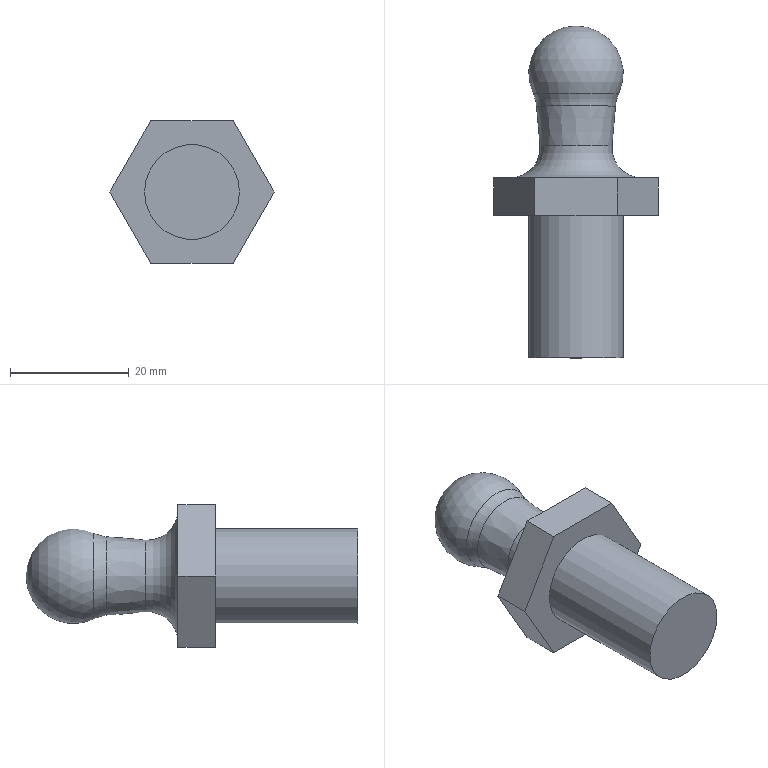Component | NX | 6 | 1 solid | 14 faces | box 27.71 x 56.01 x 24 mm | volume 11764 mm3 | plane 9 | torus 2 | cone 1 | cylinder 1 | sphere 1 | commonest cylinder face diameters 16 x1
STEP:
#1=CARTESIAN_POINT('',(0.,0.,0.));
#2=DIRECTION('',(0.,0.,1.));
#3=DIRECTION('',(1.,0.,0.));
#4=AXIS2_PLACEMENT_3D('',#1,#2,#3);
#5=CARTESIAN_POINT('',(289.409,19.836,20.));
#6=VERTEX_POINT('',#5);
#7=CARTESIAN_POINT('',(283.333,19.836,20.));
#8=DIRECTION('',(0.,1.,0.));
#9=DIRECTION('',(1.,0.,0.));
#10=AXIS2_PLACEMENT_3D('',#7,#8,#9);
#11=CIRCLE('',#10,6.076);
#12=CARTESIAN_POINT('',(283.333,31.438,20.));
#13=DIRECTION('',(0.,1.,0.));
#14=DIRECTION('',(1.,0.,0.));
#15=AXIS2_PLACEMENT_3D('',#12,#13,#14);
#16=CONICAL_SURFACE('',#15,7.091,0.08727);
#17=CARTESIAN_POINT('',(0.,-11.602));
#18=DIRECTION('',(1.,0.));
#19=VECTOR('',#18,1.);
#20=LINE('',#17,#19);
#21=(GEOMETRIC_REPRESENTATION_CONTEXT(2)PARAMETRIC_REPRESENTATION_CONTEXT()REPRESENTATION_CONTEXT('',''));
#22=DEFINITIONAL_REPRESENTATION('',(#20),#21);
#23=PCURVE('',#16,#22);
#24=CARTESIAN_POINT('',(283.333,19.4,20.));
#25=DIRECTION('',(0.,1.,0.));
#26=DIRECTION('',(1.,0.,0.));
#27=AXIS2_PLACEMENT_3D('',#24,#25,#26);
#28=TOROIDAL_SURFACE('',#27,11.057,5.);
#29=CARTESIAN_POINT('',(0.,3.054));
#30=DIRECTION('',(1.,0.));
#31=VECTOR('',#30,1.);
#32=LINE('',#29,#31);
#33=(GEOMETRIC_REPRESENTATION_CONTEXT(2)PARAMETRIC_REPRESENTATION_CONTEXT()REPRESENTATION_CONTEXT('',''));
#34=DEFINITIONAL_REPRESENTATION('',(#32),#33);
#35=PCURVE('',#28,#34);
#36=SURFACE_CURVE('',#11,(#23,#35),.PCURVE_S1.);
#37=EDGE_CURVE('',#6,#6,#36,.T.);
#38=ORIENTED_EDGE('',*,*,#37,.T.);
#39=CARTESIAN_POINT('',(289.992,26.5,20.));
#40=VERTEX_POINT('',#39);
#41=CARTESIAN_POINT('',(289.409,19.836,20.));
#42=CARTESIAN_POINT('',(289.992,26.5,20.));
#43=B_SPLINE_CURVE_WITH_KNOTS('',1,(#41,#42),.UNSPECIFIED.,.F.,.F.,(2,2),(-11.646,-4.956),.PIECEWISE_BEZIER_KNOTS.);
#44=CARTESIAN_POINT('',(6.283,0.));
#45=DIRECTION('',(0.,1.));
#46=VECTOR('',#45,1.);
#47=LINE('',#44,#46);
#48=(GEOMETRIC_REPRESENTATION_CONTEXT(2)PARAMETRIC_REPRESENTATION_CONTEXT()REPRESENTATION_CONTEXT('',''));
#49=DEFINITIONAL_REPRESENTATION('',(#47),#48);
#50=PCURVE('',#16,#49);
#51=CARTESIAN_POINT('',(0.,0.));
#52=DIRECTION('',(0.,1.));
#53=VECTOR('',#52,1.);
#54=LINE('',#51,#53);
#55=(GEOMETRIC_REPRESENTATION_CONTEXT(2)PARAMETRIC_REPRESENTATION_CONTEXT()REPRESENTATION_CONTEXT('',''));
#56=DEFINITIONAL_REPRESENTATION('',(#54),#55);
#57=PCURVE('',#16,#56);
#58=SEAM_CURVE('',#43,(#50,#57),.PCURVE_S1.);
#59=EDGE_CURVE('',#6,#40,#58,.T.);
#60=ORIENTED_EDGE('',*,*,#59,.T.);
#61=CARTESIAN_POINT('',(276.675,26.5,20.));
#62=VERTEX_POINT('',#61);
#63=CARTESIAN_POINT('',(283.333,26.5,20.));
#64=DIRECTION('',(0.,-1.,0.));
#65=DIRECTION('',(-1.,0.,0.));
#66=AXIS2_PLACEMENT_3D('',#63,#64,#65);
#67=CIRCLE('',#66,6.659);
#68=CARTESIAN_POINT('',(9.425,-4.938));
#69=DIRECTION('',(-1.,0.));
#70=VECTOR('',#69,1.);
#71=LINE('',#68,#70);
#72=(GEOMETRIC_REPRESENTATION_CONTEXT(2)PARAMETRIC_REPRESENTATION_CONTEXT()REPRESENTATION_CONTEXT('',''));
#73=DEFINITIONAL_REPRESENTATION('',(#71),#72);
#74=PCURVE('',#16,#73);
#75=CARTESIAN_POINT('',(283.333,25.977,20.));
#76=DIRECTION('',(0.,1.,0.));
#77=DIRECTION('',(1.,0.,0.));
#78=AXIS2_PLACEMENT_3D('',#75,#76,#77);
#79=TOROIDAL_SURFACE('',#78,12.636,6.);
#80=CARTESIAN_POINT('',(9.425,9.338));
#81=DIRECTION('',(-1.,0.));
#82=VECTOR('',#81,1.);
#83=LINE('',#80,#82);
#84=(GEOMETRIC_REPRESENTATION_CONTEXT(2)PARAMETRIC_REPRESENTATION_CONTEXT()REPRESENTATION_CONTEXT('',''));
#85=DEFINITIONAL_REPRESENTATION('',(#83),#84);
#86=PCURVE('',#79,#85);
#87=SURFACE_CURVE('',#67,(#74,#86),.PCURVE_S1.);
#88=EDGE_CURVE('',#40,#62,#87,.T.);
#89=ORIENTED_EDGE('',*,*,#88,.T.);
#90=CARTESIAN_POINT('',(283.333,26.5,20.));
#91=DIRECTION('',(0.,-1.,0.));
#92=DIRECTION('',(-1.,0.,0.));
#93=AXIS2_PLACEMENT_3D('',#90,#91,#92);
#94=CIRCLE('',#93,6.659);
#95=CARTESIAN_POINT('',(3.142,-4.938));
#96=DIRECTION('',(-1.,0.));
#97=VECTOR('',#96,1.);
#98=LINE('',#95,#97);
#99=(GEOMETRIC_REPRESENTATION_CONTEXT(2)PARAMETRIC_REPRESENTATION_CONTEXT()REPRESENTATION_CONTEXT('',''));
#100=DEFINITIONAL_REPRESENTATION('',(#98),#99);
#101=PCURVE('',#16,#100);
#102=CARTESIAN_POINT('',(3.142,9.338));
#103=DIRECTION('',(-1.,0.));
#104=VECTOR('',#103,1.);
#105=LINE('',#102,#104);
#106=(GEOMETRIC_REPRESENTATION_CONTEXT(2)PARAMETRIC_REPRESENTATION_CONTEXT()REPRESENTATION_CONTEXT('',''));
#107=DEFINITIONAL_REPRESENTATION('',(#105),#106);
#108=PCURVE('',#79,#107);
#109=SURFACE_CURVE('',#94,(#101,#108),.PCURVE_S1.);
#110=EDGE_CURVE('',#62,#40,#109,.T.);
#111=ORIENTED_EDGE('',*,*,#110,.T.);
#112=ORIENTED_EDGE('',*,*,#59,.F.);
#113=EDGE_LOOP('',(#38,#60,#89,#111,#112));
#114=FACE_BOUND('',#113,.T.);
#115=ADVANCED_FACE('',(#114),#16,.T.);
#116=CARTESIAN_POINT('',(291.333,8.,20.));
#117=VERTEX_POINT('',#116);
#118=CARTESIAN_POINT('',(283.333,8.,20.));
#119=DIRECTION('',(0.,1.,0.));
#120=DIRECTION('',(1.,0.,0.));
#121=AXIS2_PLACEMENT_3D('',#118,#119,#120);
#122=CIRCLE('',#121,8.);
#123=CARTESIAN_POINT('',(283.333,8.,20.));
#124=DIRECTION('',(0.,-1.,0.));
#125=DIRECTION('',(-1.,0.,0.));
#126=AXIS2_PLACEMENT_3D('',#123,#124,#125);
#127=CYLINDRICAL_SURFACE('',#126,8.);
#128=CARTESIAN_POINT('',(9.425,0.));
#129=DIRECTION('',(-1.,0.));
#130=VECTOR('',#129,1.);
#131=LINE('',#128,#130);
#132=(GEOMETRIC_REPRESENTATION_CONTEXT(2)PARAMETRIC_REPRESENTATION_CONTEXT()REPRESENTATION_CONTEXT('',''));
#133=DEFINITIONAL_REPRESENTATION('',(#131),#132);
#134=PCURVE('',#127,#133);
#135=CARTESIAN_POINT('',(283.333,8.,20.));
#136=DIRECTION('',(0.,1.,0.));
#137=DIRECTION('',(1.,0.,0.));
#138=AXIS2_PLACEMENT_3D('',#135,#136,#137);
#139=PLANE('',#138);
#140=CARTESIAN_POINT('',(0.,0.));
#141=DIRECTION('',(1.,0.));
#142=AXIS2_PLACEMENT_2D('',#140,#141);
#143=CIRCLE('',#142,8.);
#144=(GEOMETRIC_REPRESENTATION_CONTEXT(2)PARAMETRIC_REPRESENTATION_CONTEXT()REPRESENTATION_CONTEXT('',''));
#145=DEFINITIONAL_REPRESENTATION('',(#143),#144);
#146=PCURVE('',#139,#145);
#147=SURFACE_CURVE('',#122,(#134,#146),.PCURVE_S1.);
#148=EDGE_CURVE('',#117,#117,#147,.T.);
#149=ORIENTED_EDGE('',*,*,#148,.F.);
#150=CARTESIAN_POINT('',(291.333,-16.,20.));
#151=VERTEX_POINT('',#150);
#152=CARTESIAN_POINT('',(291.333,8.,20.));
#153=CARTESIAN_POINT('',(291.333,-16.,20.));
#154=B_SPLINE_CURVE_WITH_KNOTS('',1,(#152,#153),.UNSPECIFIED.,.F.,.F.,(2,2),(0.,24.),.PIECEWISE_BEZIER_KNOTS.);
#155=CARTESIAN_POINT('',(9.425,0.));
#156=DIRECTION('',(0.,1.));
#157=VECTOR('',#156,1.);
#158=LINE('',#155,#157);
#159=(GEOMETRIC_REPRESENTATION_CONTEXT(2)PARAMETRIC_REPRESENTATION_CONTEXT()REPRESENTATION_CONTEXT('',''));
#160=DEFINITIONAL_REPRESENTATION('',(#158),#159);
#161=PCURVE('',#127,#160);
#162=CARTESIAN_POINT('',(3.142,0.));
#163=DIRECTION('',(0.,1.));
#164=VECTOR('',#163,1.);
#165=LINE('',#162,#164);
#166=(GEOMETRIC_REPRESENTATION_CONTEXT(2)PARAMETRIC_REPRESENTATION_CONTEXT()REPRESENTATION_CONTEXT('',''));
#167=DEFINITIONAL_REPRESENTATION('',(#165),#166);
#168=PCURVE('',#127,#167);
#169=SEAM_CURVE('',#154,(#161,#168),.PCURVE_S1.);
#170=EDGE_CURVE('',#117,#151,#169,.T.);
#171=ORIENTED_EDGE('',*,*,#170,.T.);
#172=CARTESIAN_POINT('',(283.333,-16.,20.));
#173=DIRECTION('',(0.,1.,0.));
#174=DIRECTION('',(1.,0.,0.));
#175=AXIS2_PLACEMENT_3D('',#172,#173,#174);
#176=CIRCLE('',#175,8.);
#177=CARTESIAN_POINT('',(9.425,24.));
#178=DIRECTION('',(-1.,0.));
#179=VECTOR('',#178,1.);
#180=LINE('',#177,#179);
#181=(GEOMETRIC_REPRESENTATION_CONTEXT(2)PARAMETRIC_REPRESENTATION_CONTEXT()REPRESENTATION_CONTEXT('',''));
#182=DEFINITIONAL_REPRESENTATION('',(#180),#181);
#183=PCURVE('',#127,#182);
#184=CARTESIAN_POINT('',(283.333,-16.,20.));
#185=DIRECTION('',(0.,1.,0.));
#186=DIRECTION('',(1.,0.,0.));
#187=AXIS2_PLACEMENT_3D('',#184,#185,#186);
#188=PLANE('',#187);
#189=CARTESIAN_POINT('',(0.,0.));
#190=DIRECTION('',(1.,0.));
#191=AXIS2_PLACEMENT_2D('',#189,#190);
#192=CIRCLE('',#191,8.);
#193=(GEOMETRIC_REPRESENTATION_CONTEXT(2)PARAMETRIC_REPRESENTATION_CONTEXT()REPRESENTATION_CONTEXT('',''));
#194=DEFINITIONAL_REPRESENTATION('',(#192),#193);
#195=PCURVE('',#188,#194);
#196=SURFACE_CURVE('',#176,(#183,#195),.PCURVE_S1.);
#197=EDGE_CURVE('',#151,#151,#196,.T.);
#198=ORIENTED_EDGE('',*,*,#197,.T.);
#199=ORIENTED_EDGE('',*,*,#170,.F.);
#200=EDGE_LOOP('',(#149,#171,#198,#199));
#201=FACE_BOUND('',#200,.T.);
#202=ADVANCED_FACE('',(#201),#127,.T.);
#203=ORIENTED_EDGE('',*,*,#197,.F.);
#204=EDGE_LOOP('',(#203));
#205=FACE_BOUND('',#204,.T.);
#206=ADVANCED_FACE('',(#205),#188,.F.);
#207=CARTESIAN_POINT('',(269.477,8.,20.));
#208=VERTEX_POINT('',#207);
#209=CARTESIAN_POINT('',(276.405,8.,32.));
#210=VERTEX_POINT('',#209);
#211=CARTESIAN_POINT('',(269.477,8.,20.));
#212=DIRECTION('',(0.5,0.,0.866));
#213=VECTOR('',#212,1.);
#214=LINE('',#211,#213);
#215=CARTESIAN_POINT('',(269.477,14.4,20.));
#216=DIRECTION('',(0.866,0.,-0.5));
#217=DIRECTION('',(-0.5,0.,-0.866));
#218=AXIS2_PLACEMENT_3D('',#215,#216,#217);
#219=PLANE('',#218);
#220=CARTESIAN_POINT('',(0.,-6.4));
#221=DIRECTION('',(-1.,0.));
#222=VECTOR('',#221,1.);
#223=LINE('',#220,#222);
#224=(GEOMETRIC_REPRESENTATION_CONTEXT(2)PARAMETRIC_REPRESENTATION_CONTEXT()REPRESENTATION_CONTEXT('',''));
#225=DEFINITIONAL_REPRESENTATION('',(#223),#224);
#226=PCURVE('',#219,#225);
#227=CARTESIAN_POINT('',(-13.856,0.));
#228=DIRECTION('',(0.5,-0.866));
#229=VECTOR('',#228,1.);
#230=LINE('',#227,#229);
#231=(GEOMETRIC_REPRESENTATION_CONTEXT(2)PARAMETRIC_REPRESENTATION_CONTEXT()REPRESENTATION_CONTEXT('',''));
#232=DEFINITIONAL_REPRESENTATION('',(#230),#231);
#233=PCURVE('',#139,#232);
#234=SURFACE_CURVE('',#214,(#226,#233),.PCURVE_S1.);
#235=EDGE_CURVE('',#208,#210,#234,.T.);
#236=ORIENTED_EDGE('',*,*,#235,.T.);
#237=CARTESIAN_POINT('',(276.405,14.4,32.));
#238=VERTEX_POINT('',#237);
#239=CARTESIAN_POINT('',(276.405,14.4,32.));
#240=DIRECTION('',(0.,-1.,0.));
#241=VECTOR('',#240,1.);
#242=LINE('',#239,#241);
#243=CARTESIAN_POINT('',(-13.856,0.));
#244=DIRECTION('',(0.,-1.));
#245=VECTOR('',#244,1.);
#246=LINE('',#243,#245);
#247=(GEOMETRIC_REPRESENTATION_CONTEXT(2)PARAMETRIC_REPRESENTATION_CONTEXT()REPRESENTATION_CONTEXT('',''));
#248=DEFINITIONAL_REPRESENTATION('',(#246),#247);
#249=PCURVE('',#219,#248);
#250=CARTESIAN_POINT('',(276.405,14.4,32.));
#251=DIRECTION('',(0.,0.,-1.));
#252=DIRECTION('',(-1.,0.,-0.));
#253=AXIS2_PLACEMENT_3D('',#250,#251,#252);
#254=PLANE('',#253);
#255=CARTESIAN_POINT('',(0.,0.));
#256=DIRECTION('',(0.,-1.));
#257=VECTOR('',#256,1.);
#258=LINE('',#255,#257);
#259=(GEOMETRIC_REPRESENTATION_CONTEXT(2)PARAMETRIC_REPRESENTATION_CONTEXT()REPRESENTATION_CONTEXT('',''));
#260=DEFINITIONAL_REPRESENTATION('',(#258),#259);
#261=PCURVE('',#254,#260);
#262=SURFACE_CURVE('',#242,(#249,#261),.PCURVE_S1.);
#263=EDGE_CURVE('',#238,#210,#262,.T.);
#264=ORIENTED_EDGE('',*,*,#263,.F.);
#265=CARTESIAN_POINT('',(269.477,14.4,20.));
#266=VERTEX_POINT('',#265);
#267=CARTESIAN_POINT('',(269.477,14.4,20.));
#268=DIRECTION('',(0.5,0.,0.866));
#269=VECTOR('',#268,1.);
#270=LINE('',#267,#269);
#271=CARTESIAN_POINT('',(0.,0.));
#272=DIRECTION('',(-1.,0.));
#273=VECTOR('',#272,1.);
#274=LINE('',#271,#273);
#275=(GEOMETRIC_REPRESENTATION_CONTEXT(2)PARAMETRIC_REPRESENTATION_CONTEXT()REPRESENTATION_CONTEXT('',''));
#276=DEFINITIONAL_REPRESENTATION('',(#274),#275);
#277=PCURVE('',#219,#276);
#278=CARTESIAN_POINT('',(283.333,14.4,20.));
#279=DIRECTION('',(0.,1.,0.));
#280=DIRECTION('',(1.,0.,0.));
#281=AXIS2_PLACEMENT_3D('',#278,#279,#280);
#282=PLANE('',#281);
#283=CARTESIAN_POINT('',(-13.856,0.));
#284=DIRECTION('',(0.5,-0.866));
#285=VECTOR('',#284,1.);
#286=LINE('',#283,#285);
#287=(GEOMETRIC_REPRESENTATION_CONTEXT(2)PARAMETRIC_REPRESENTATION_CONTEXT()REPRESENTATION_CONTEXT('',''));
#288=DEFINITIONAL_REPRESENTATION('',(#286),#287);
#289=PCURVE('',#282,#288);
#290=SURFACE_CURVE('',#270,(#277,#289),.PCURVE_S1.);
#291=EDGE_CURVE('',#266,#238,#290,.T.);
#292=ORIENTED_EDGE('',*,*,#291,.F.);
#293=CARTESIAN_POINT('',(269.477,14.4,20.));
#294=DIRECTION('',(0.,-1.,0.));
#295=VECTOR('',#294,1.);
#296=LINE('',#293,#295);
#297=CARTESIAN_POINT('',(0.,0.));
#298=DIRECTION('',(0.,-1.));
#299=VECTOR('',#298,1.);
#300=LINE('',#297,#299);
#301=(GEOMETRIC_REPRESENTATION_CONTEXT(2)PARAMETRIC_REPRESENTATION_CONTEXT()REPRESENTATION_CONTEXT('',''));
#302=DEFINITIONAL_REPRESENTATION('',(#300),#301);
#303=PCURVE('',#219,#302);
#304=CARTESIAN_POINT('',(276.405,14.4,8.));
#305=DIRECTION('',(0.866,0.,0.5));
#306=DIRECTION('',(0.5,0.,-0.866));
#307=AXIS2_PLACEMENT_3D('',#304,#305,#306);
#308=PLANE('',#307);
#309=CARTESIAN_POINT('',(-13.856,0.));
#310=DIRECTION('',(0.,-1.));
#311=VECTOR('',#310,1.);
#312=LINE('',#309,#311);
#313=(GEOMETRIC_REPRESENTATION_CONTEXT(2)PARAMETRIC_REPRESENTATION_CONTEXT()REPRESENTATION_CONTEXT('',''));
#314=DEFINITIONAL_REPRESENTATION('',(#312),#313);
#315=PCURVE('',#308,#314);
#316=SURFACE_CURVE('',#296,(#303,#315),.PCURVE_S1.);
#317=EDGE_CURVE('',#266,#208,#316,.T.);
#318=ORIENTED_EDGE('',*,*,#317,.T.);
#319=EDGE_LOOP('',(#236,#264,#292,#318));
#320=FACE_BOUND('',#319,.T.);
#321=ADVANCED_FACE('',(#320),#219,.F.);
#322=CARTESIAN_POINT('',(290.262,8.,32.));
#323=VERTEX_POINT('',#322);
#324=CARTESIAN_POINT('',(276.405,8.,32.));
#325=DIRECTION('',(1.,0.,0.));
#326=VECTOR('',#325,1.);
#327=LINE('',#324,#326);
#328=CARTESIAN_POINT('',(0.,-6.4));
#329=DIRECTION('',(-1.,0.));
#330=VECTOR('',#329,1.);
#331=LINE('',#328,#330);
#332=(GEOMETRIC_REPRESENTATION_CONTEXT(2)PARAMETRIC_REPRESENTATION_CONTEXT()REPRESENTATION_CONTEXT('',''));
#333=DEFINITIONAL_REPRESENTATION('',(#331),#332);
#334=PCURVE('',#254,#333);
#335=CARTESIAN_POINT('',(-6.928,-12.));
#336=DIRECTION('',(1.,-0.));
#337=VECTOR('',#336,1.);
#338=LINE('',#335,#337);
#339=(GEOMETRIC_REPRESENTATION_CONTEXT(2)PARAMETRIC_REPRESENTATION_CONTEXT()REPRESENTATION_CONTEXT('',''));
#340=DEFINITIONAL_REPRESENTATION('',(#338),#339);
#341=PCURVE('',#139,#340);
#342=SURFACE_CURVE('',#327,(#334,#341),.PCURVE_S1.);
#343=EDGE_CURVE('',#210,#323,#342,.T.);
#344=ORIENTED_EDGE('',*,*,#343,.T.);
#345=CARTESIAN_POINT('',(290.262,14.4,32.));
#346=VERTEX_POINT('',#345);
#347=CARTESIAN_POINT('',(290.262,14.4,32.));
#348=DIRECTION('',(0.,-1.,0.));
#349=VECTOR('',#348,1.);
#350=LINE('',#347,#349);
#351=CARTESIAN_POINT('',(-13.856,0.));
#352=DIRECTION('',(0.,-1.));
#353=VECTOR('',#352,1.);
#354=LINE('',#351,#353);
#355=(GEOMETRIC_REPRESENTATION_CONTEXT(2)PARAMETRIC_REPRESENTATION_CONTEXT()REPRESENTATION_CONTEXT('',''));
#356=DEFINITIONAL_REPRESENTATION('',(#354),#355);
#357=PCURVE('',#254,#356);
#358=CARTESIAN_POINT('',(290.262,14.4,32.));
#359=DIRECTION('',(-0.866,0.,-0.5));
#360=DIRECTION('',(-0.5,0.,0.866));
#361=AXIS2_PLACEMENT_3D('',#358,#359,#360);
#362=PLANE('',#361);
#363=CARTESIAN_POINT('',(0.,0.));
#364=DIRECTION('',(0.,-1.));
#365=VECTOR('',#364,1.);
#366=LINE('',#363,#365);
#367=(GEOMETRIC_REPRESENTATION_CONTEXT(2)PARAMETRIC_REPRESENTATION_CONTEXT()REPRESENTATION_CONTEXT('',''));
#368=DEFINITIONAL_REPRESENTATION('',(#366),#367);
#369=PCURVE('',#362,#368);
#370=SURFACE_CURVE('',#350,(#357,#369),.PCURVE_S1.);
#371=EDGE_CURVE('',#346,#323,#370,.T.);
#372=ORIENTED_EDGE('',*,*,#371,.F.);
#373=CARTESIAN_POINT('',(276.405,14.4,32.));
#374=DIRECTION('',(1.,0.,0.));
#375=VECTOR('',#374,1.);
#376=LINE('',#373,#375);
#377=CARTESIAN_POINT('',(0.,0.));
#378=DIRECTION('',(-1.,0.));
#379=VECTOR('',#378,1.);
#380=LINE('',#377,#379);
#381=(GEOMETRIC_REPRESENTATION_CONTEXT(2)PARAMETRIC_REPRESENTATION_CONTEXT()REPRESENTATION_CONTEXT('',''));
#382=DEFINITIONAL_REPRESENTATION('',(#380),#381);
#383=PCURVE('',#254,#382);
#384=CARTESIAN_POINT('',(-6.928,-12.));
#385=DIRECTION('',(1.,-0.));
#386=VECTOR('',#385,1.);
#387=LINE('',#384,#386);
#388=(GEOMETRIC_REPRESENTATION_CONTEXT(2)PARAMETRIC_REPRESENTATION_CONTEXT()REPRESENTATION_CONTEXT('',''));
#389=DEFINITIONAL_REPRESENTATION('',(#387),#388);
#390=PCURVE('',#282,#389);
#391=SURFACE_CURVE('',#376,(#383,#390),.PCURVE_S1.);
#392=EDGE_CURVE('',#238,#346,#391,.T.);
#393=ORIENTED_EDGE('',*,*,#392,.F.);
#394=ORIENTED_EDGE('',*,*,#263,.T.);
#395=EDGE_LOOP('',(#344,#372,#393,#394));
#396=FACE_BOUND('',#395,.T.);
#397=ADVANCED_FACE('',(#396),#254,.F.);
#398=CARTESIAN_POINT('',(297.19,8.,20.));
#399=VERTEX_POINT('',#398);
#400=CARTESIAN_POINT('',(290.262,8.,32.));
#401=DIRECTION('',(0.5,0.,-0.866));
#402=VECTOR('',#401,1.);
#403=LINE('',#400,#402);
#404=CARTESIAN_POINT('',(0.,-6.4));
#405=DIRECTION('',(-1.,0.));
#406=VECTOR('',#405,1.);
#407=LINE('',#404,#406);
#408=(GEOMETRIC_REPRESENTATION_CONTEXT(2)PARAMETRIC_REPRESENTATION_CONTEXT()REPRESENTATION_CONTEXT('',''));
#409=DEFINITIONAL_REPRESENTATION('',(#407),#408);
#410=PCURVE('',#362,#409);
#411=CARTESIAN_POINT('',(6.928,-12.));
#412=DIRECTION('',(0.5,0.866));
#413=VECTOR('',#412,1.);
#414=LINE('',#411,#413);
#415=(GEOMETRIC_REPRESENTATION_CONTEXT(2)PARAMETRIC_REPRESENTATION_CONTEXT()REPRESENTATION_CONTEXT('',''));
#416=DEFINITIONAL_REPRESENTATION('',(#414),#415);
#417=PCURVE('',#139,#416);
#418=SURFACE_CURVE('',#403,(#410,#417),.PCURVE_S1.);
#419=EDGE_CURVE('',#323,#399,#418,.T.);
#420=ORIENTED_EDGE('',*,*,#419,.T.);
#421=CARTESIAN_POINT('',(297.19,14.4,20.));
#422=VERTEX_POINT('',#421);
#423=CARTESIAN_POINT('',(297.19,14.4,20.));
#424=DIRECTION('',(0.,-1.,0.));
#425=VECTOR('',#424,1.);
#426=LINE('',#423,#425);
#427=CARTESIAN_POINT('',(-13.856,0.));
#428=DIRECTION('',(0.,-1.));
#429=VECTOR('',#428,1.);
#430=LINE('',#427,#429);
#431=(GEOMETRIC_REPRESENTATION_CONTEXT(2)PARAMETRIC_REPRESENTATION_CONTEXT()REPRESENTATION_CONTEXT('',''));
#432=DEFINITIONAL_REPRESENTATION('',(#430),#431);
#433=PCURVE('',#362,#432);
#434=CARTESIAN_POINT('',(297.19,14.4,20.));
#435=DIRECTION('',(-0.866,0.,0.5));
#436=DIRECTION('',(0.5,0.,0.866));
#437=AXIS2_PLACEMENT_3D('',#434,#435,#436);
#438=PLANE('',#437);
#439=CARTESIAN_POINT('',(0.,0.));
#440=DIRECTION('',(0.,-1.));
#441=VECTOR('',#440,1.);
#442=LINE('',#439,#441);
#443=(GEOMETRIC_REPRESENTATION_CONTEXT(2)PARAMETRIC_REPRESENTATION_CONTEXT()REPRESENTATION_CONTEXT('',''));
#444=DEFINITIONAL_REPRESENTATION('',(#442),#443);
#445=PCURVE('',#438,#444);
#446=SURFACE_CURVE('',#426,(#433,#445),.PCURVE_S1.);
#447=EDGE_CURVE('',#422,#399,#446,.T.);
#448=ORIENTED_EDGE('',*,*,#447,.F.);
#449=CARTESIAN_POINT('',(290.262,14.4,32.));
#450=DIRECTION('',(0.5,0.,-0.866));
#451=VECTOR('',#450,1.);
#452=LINE('',#449,#451);
#453=CARTESIAN_POINT('',(0.,0.));
#454=DIRECTION('',(-1.,0.));
#455=VECTOR('',#454,1.);
#456=LINE('',#453,#455);
#457=(GEOMETRIC_REPRESENTATION_CONTEXT(2)PARAMETRIC_REPRESENTATION_CONTEXT()REPRESENTATION_CONTEXT('',''));
#458=DEFINITIONAL_REPRESENTATION('',(#456),#457);
#459=PCURVE('',#362,#458);
#460=CARTESIAN_POINT('',(6.928,-12.));
#461=DIRECTION('',(0.5,0.866));
#462=VECTOR('',#461,1.);
#463=LINE('',#460,#462);
#464=(GEOMETRIC_REPRESENTATION_CONTEXT(2)PARAMETRIC_REPRESENTATION_CONTEXT()REPRESENTATION_CONTEXT('',''));
#465=DEFINITIONAL_REPRESENTATION('',(#463),#464);
#466=PCURVE('',#282,#465);
#467=SURFACE_CURVE('',#452,(#459,#466),.PCURVE_S1.);
#468=EDGE_CURVE('',#346,#422,#467,.T.);
#469=ORIENTED_EDGE('',*,*,#468,.F.);
#470=ORIENTED_EDGE('',*,*,#371,.T.);
#471=EDGE_LOOP('',(#420,#448,#469,#470));
#472=FACE_BOUND('',#471,.T.);
#473=ADVANCED_FACE('',(#472),#362,.F.);
#474=CARTESIAN_POINT('',(290.262,8.,8.));
#475=VERTEX_POINT('',#474);
#476=CARTESIAN_POINT('',(297.19,8.,20.));
#477=DIRECTION('',(-0.5,0.,-0.866));
#478=VECTOR('',#477,1.);
#479=LINE('',#476,#478);
#480=CARTESIAN_POINT('',(0.,-6.4));
#481=DIRECTION('',(-1.,0.));
#482=VECTOR('',#481,1.);
#483=LINE('',#480,#482);
#484=(GEOMETRIC_REPRESENTATION_CONTEXT(2)PARAMETRIC_REPRESENTATION_CONTEXT()REPRESENTATION_CONTEXT('',''));
#485=DEFINITIONAL_REPRESENTATION('',(#483),#484);
#486=PCURVE('',#438,#485);
#487=CARTESIAN_POINT('',(13.856,-0.));
#488=DIRECTION('',(-0.5,0.866));
#489=VECTOR('',#488,1.);
#490=LINE('',#487,#489);
#491=(GEOMETRIC_REPRESENTATION_CONTEXT(2)PARAMETRIC_REPRESENTATION_CONTEXT()REPRESENTATION_CONTEXT('',''));
#492=DEFINITIONAL_REPRESENTATION('',(#490),#491);
#493=PCURVE('',#139,#492);
#494=SURFACE_CURVE('',#479,(#486,#493),.PCURVE_S1.);
#495=EDGE_CURVE('',#399,#475,#494,.T.);
#496=ORIENTED_EDGE('',*,*,#495,.T.);
#497=CARTESIAN_POINT('',(290.262,14.4,8.));
#498=VERTEX_POINT('',#497);
#499=CARTESIAN_POINT('',(290.262,14.4,8.));
#500=DIRECTION('',(0.,-1.,0.));
#501=VECTOR('',#500,1.);
#502=LINE('',#499,#501);
#503=CARTESIAN_POINT('',(-13.856,0.));
#504=DIRECTION('',(0.,-1.));
#505=VECTOR('',#504,1.);
#506=LINE('',#503,#505);
#507=(GEOMETRIC_REPRESENTATION_CONTEXT(2)PARAMETRIC_REPRESENTATION_CONTEXT()REPRESENTATION_CONTEXT('',''));
#508=DEFINITIONAL_REPRESENTATION('',(#506),#507);
#509=PCURVE('',#438,#508);
#510=CARTESIAN_POINT('',(290.262,14.4,8.));
#511=DIRECTION('',(-0.,0.,1.));
#512=DIRECTION('',(1.,0.,0.));
#513=AXIS2_PLACEMENT_3D('',#510,#511,#512);
#514=PLANE('',#513);
#515=CARTESIAN_POINT('',(0.,0.));
#516=DIRECTION('',(0.,-1.));
#517=VECTOR('',#516,1.);
#518=LINE('',#515,#517);
#519=(GEOMETRIC_REPRESENTATION_CONTEXT(2)PARAMETRIC_REPRESENTATION_CONTEXT()REPRESENTATION_CONTEXT('',''));
#520=DEFINITIONAL_REPRESENTATION('',(#518),#519);
#521=PCURVE('',#514,#520);
#522=SURFACE_CURVE('',#502,(#509,#521),.PCURVE_S1.);
#523=EDGE_CURVE('',#498,#475,#522,.T.);
#524=ORIENTED_EDGE('',*,*,#523,.F.);
#525=CARTESIAN_POINT('',(297.19,14.4,20.));
#526=DIRECTION('',(-0.5,0.,-0.866));
#527=VECTOR('',#526,1.);
#528=LINE('',#525,#527);
#529=CARTESIAN_POINT('',(0.,0.));
#530=DIRECTION('',(-1.,0.));
#531=VECTOR('',#530,1.);
#532=LINE('',#529,#531);
#533=(GEOMETRIC_REPRESENTATION_CONTEXT(2)PARAMETRIC_REPRESENTATION_CONTEXT()REPRESENTATION_CONTEXT('',''));
#534=DEFINITIONAL_REPRESENTATION('',(#532),#533);
#535=PCURVE('',#438,#534);
#536=CARTESIAN_POINT('',(13.856,-0.));
#537=DIRECTION('',(-0.5,0.866));
#538=VECTOR('',#537,1.);
#539=LINE('',#536,#538);
#540=(GEOMETRIC_REPRESENTATION_CONTEXT(2)PARAMETRIC_REPRESENTATION_CONTEXT()REPRESENTATION_CONTEXT('',''));
#541=DEFINITIONAL_REPRESENTATION('',(#539),#540);
#542=PCURVE('',#282,#541);
#543=SURFACE_CURVE('',#528,(#535,#542),.PCURVE_S1.);
#544=EDGE_CURVE('',#422,#498,#543,.T.);
#545=ORIENTED_EDGE('',*,*,#544,.F.);
#546=ORIENTED_EDGE('',*,*,#447,.T.);
#547=EDGE_LOOP('',(#496,#524,#545,#546));
#548=FACE_BOUND('',#547,.T.);
#549=ADVANCED_FACE('',(#548),#438,.F.);
#550=CARTESIAN_POINT('',(276.405,8.,8.));
#551=VERTEX_POINT('',#550);
#552=CARTESIAN_POINT('',(290.262,8.,8.));
#553=DIRECTION('',(-1.,0.,-0.));
#554=VECTOR('',#553,1.);
#555=LINE('',#552,#554);
#556=CARTESIAN_POINT('',(0.,-6.4));
#557=DIRECTION('',(-1.,0.));
#558=VECTOR('',#557,1.);
#559=LINE('',#556,#558);
#560=(GEOMETRIC_REPRESENTATION_CONTEXT(2)PARAMETRIC_REPRESENTATION_CONTEXT()REPRESENTATION_CONTEXT('',''));
#561=DEFINITIONAL_REPRESENTATION('',(#559),#560);
#562=PCURVE('',#514,#561);
#563=CARTESIAN_POINT('',(6.928,12.));
#564=DIRECTION('',(-1.,0.));
#565=VECTOR('',#564,1.);
#566=LINE('',#563,#565);
#567=(GEOMETRIC_REPRESENTATION_CONTEXT(2)PARAMETRIC_REPRESENTATION_CONTEXT()REPRESENTATION_CONTEXT('',''));
#568=DEFINITIONAL_REPRESENTATION('',(#566),#567);
#569=PCURVE('',#139,#568);
#570=SURFACE_CURVE('',#555,(#562,#569),.PCURVE_S1.);
#571=EDGE_CURVE('',#475,#551,#570,.T.);
#572=ORIENTED_EDGE('',*,*,#571,.T.);
#573=CARTESIAN_POINT('',(276.405,14.4,8.));
#574=VERTEX_POINT('',#573);
#575=CARTESIAN_POINT('',(276.405,14.4,8.));
#576=DIRECTION('',(0.,-1.,0.));
#577=VECTOR('',#576,1.);
#578=LINE('',#575,#577);
#579=CARTESIAN_POINT('',(-13.856,0.));
#580=DIRECTION('',(0.,-1.));
#581=VECTOR('',#580,1.);
#582=LINE('',#579,#581);
#583=(GEOMETRIC_REPRESENTATION_CONTEXT(2)PARAMETRIC_REPRESENTATION_CONTEXT()REPRESENTATION_CONTEXT('',''));
#584=DEFINITIONAL_REPRESENTATION('',(#582),#583);
#585=PCURVE('',#514,#584);
#586=CARTESIAN_POINT('',(0.,0.));
#587=DIRECTION('',(0.,-1.));
#588=VECTOR('',#587,1.);
#589=LINE('',#586,#588);
#590=(GEOMETRIC_REPRESENTATION_CONTEXT(2)PARAMETRIC_REPRESENTATION_CONTEXT()REPRESENTATION_CONTEXT('',''));
#591=DEFINITIONAL_REPRESENTATION('',(#589),#590);
#592=PCURVE('',#308,#591);
#593=SURFACE_CURVE('',#578,(#585,#592),.PCURVE_S1.);
#594=EDGE_CURVE('',#574,#551,#593,.T.);
#595=ORIENTED_EDGE('',*,*,#594,.F.);
#596=CARTESIAN_POINT('',(290.262,14.4,8.));
#597=DIRECTION('',(-1.,0.,-0.));
#598=VECTOR('',#597,1.);
#599=LINE('',#596,#598);
#600=CARTESIAN_POINT('',(0.,0.));
#601=DIRECTION('',(-1.,0.));
#602=VECTOR('',#601,1.);
#603=LINE('',#600,#602);
#604=(GEOMETRIC_REPRESENTATION_CONTEXT(2)PARAMETRIC_REPRESENTATION_CONTEXT()REPRESENTATION_CONTEXT('',''));
#605=DEFINITIONAL_REPRESENTATION('',(#603),#604);
#606=PCURVE('',#514,#605);
#607=CARTESIAN_POINT('',(6.928,12.));
#608=DIRECTION('',(-1.,0.));
#609=VECTOR('',#608,1.);
#610=LINE('',#607,#609);
#611=(GEOMETRIC_REPRESENTATION_CONTEXT(2)PARAMETRIC_REPRESENTATION_CONTEXT()REPRESENTATION_CONTEXT('',''));
#612=DEFINITIONAL_REPRESENTATION('',(#610),#611);
#613=PCURVE('',#282,#612);
#614=SURFACE_CURVE('',#599,(#606,#613),.PCURVE_S1.);
#615=EDGE_CURVE('',#498,#574,#614,.T.);
#616=ORIENTED_EDGE('',*,*,#615,.F.);
#617=ORIENTED_EDGE('',*,*,#523,.T.);
#618=EDGE_LOOP('',(#572,#595,#616,#617));
#619=FACE_BOUND('',#618,.T.);
#620=ADVANCED_FACE('',(#619),#514,.F.);
#621=CARTESIAN_POINT('',(276.405,8.,8.));
#622=DIRECTION('',(-0.5,0.,0.866));
#623=VECTOR('',#622,1.);
#624=LINE('',#621,#623);
#625=CARTESIAN_POINT('',(0.,-6.4));
#626=DIRECTION('',(-1.,0.));
#627=VECTOR('',#626,1.);
#628=LINE('',#625,#627);
#629=(GEOMETRIC_REPRESENTATION_CONTEXT(2)PARAMETRIC_REPRESENTATION_CONTEXT()REPRESENTATION_CONTEXT('',''));
#630=DEFINITIONAL_REPRESENTATION('',(#628),#629);
#631=PCURVE('',#308,#630);
#632=CARTESIAN_POINT('',(-6.928,12.));
#633=DIRECTION('',(-0.5,-0.866));
#634=VECTOR('',#633,1.);
#635=LINE('',#632,#634);
#636=(GEOMETRIC_REPRESENTATION_CONTEXT(2)PARAMETRIC_REPRESENTATION_CONTEXT()REPRESENTATION_CONTEXT('',''));
#637=DEFINITIONAL_REPRESENTATION('',(#635),#636);
#638=PCURVE('',#139,#637);
#639=SURFACE_CURVE('',#624,(#631,#638),.PCURVE_S1.);
#640=EDGE_CURVE('',#551,#208,#639,.T.);
#641=ORIENTED_EDGE('',*,*,#640,.T.);
#642=ORIENTED_EDGE('',*,*,#317,.F.);
#643=CARTESIAN_POINT('',(276.405,14.4,8.));
#644=DIRECTION('',(-0.5,0.,0.866));
#645=VECTOR('',#644,1.);
#646=LINE('',#643,#645);
#647=CARTESIAN_POINT('',(0.,0.));
#648=DIRECTION('',(-1.,0.));
#649=VECTOR('',#648,1.);
#650=LINE('',#647,#649);
#651=(GEOMETRIC_REPRESENTATION_CONTEXT(2)PARAMETRIC_REPRESENTATION_CONTEXT()REPRESENTATION_CONTEXT('',''));
#652=DEFINITIONAL_REPRESENTATION('',(#650),#651);
#653=PCURVE('',#308,#652);
#654=CARTESIAN_POINT('',(-6.928,12.));
#655=DIRECTION('',(-0.5,-0.866));
#656=VECTOR('',#655,1.);
#657=LINE('',#654,#656);
#658=(GEOMETRIC_REPRESENTATION_CONTEXT(2)PARAMETRIC_REPRESENTATION_CONTEXT()REPRESENTATION_CONTEXT('',''));
#659=DEFINITIONAL_REPRESENTATION('',(#657),#658);
#660=PCURVE('',#282,#659);
#661=SURFACE_CURVE('',#646,(#653,#660),.PCURVE_S1.);
#662=EDGE_CURVE('',#574,#266,#661,.T.);
#663=ORIENTED_EDGE('',*,*,#662,.F.);
#664=ORIENTED_EDGE('',*,*,#594,.T.);
#665=EDGE_LOOP('',(#641,#642,#663,#664));
#666=FACE_BOUND('',#665,.T.);
#667=ADVANCED_FACE('',(#666),#308,.F.);
#668=CARTESIAN_POINT('',(294.39,14.4,20.));
#669=VERTEX_POINT('',#668);
#670=CARTESIAN_POINT('',(283.333,14.4,20.));
#671=DIRECTION('',(0.,-1.,0.));
#672=DIRECTION('',(1.,0.,0.));
#673=AXIS2_PLACEMENT_3D('',#670,#671,#672);
#674=CIRCLE('',#673,11.057);
#675=CARTESIAN_POINT('',(11.057,0.));
#676=CARTESIAN_POINT('',(11.057,-19.15));
#677=CARTESIAN_POINT('',(-5.528,-9.575));
#678=CARTESIAN_POINT('',(-22.113,-0.));
#679=CARTESIAN_POINT('',(-5.528,9.575));
#680=CARTESIAN_POINT('',(11.057,19.15));
#681=CARTESIAN_POINT('',(11.057,0.));
#682=(BOUNDED_CURVE()B_SPLINE_CURVE(2,(#675,#676,#677,#678,#679,#680,#681),.UNSPECIFIED.,.T.,.F.)B_SPLINE_CURVE_WITH_KNOTS((1,2,2,2,2,1),(-2.094,0.,2.094,4.189,6.283,8.378),.UNSPECIFIED.)CURVE()GEOMETRIC_REPRESENTATION_ITEM()RATIONAL_B_SPLINE_CURVE((1.,0.5,1.,0.5,1.,0.5,1.))REPRESENTATION_ITEM(''));
#683=(GEOMETRIC_REPRESENTATION_CONTEXT(2)PARAMETRIC_REPRESENTATION_CONTEXT()REPRESENTATION_CONTEXT('',''));
#684=DEFINITIONAL_REPRESENTATION('',(#682),#683);
#685=PCURVE('',#282,#684);
#686=CARTESIAN_POINT('',(6.283,4.712));
#687=DIRECTION('',(-1.,0.));
#688=VECTOR('',#687,1.);
#689=LINE('',#686,#688);
#690=(GEOMETRIC_REPRESENTATION_CONTEXT(2)PARAMETRIC_REPRESENTATION_CONTEXT()REPRESENTATION_CONTEXT('',''));
#691=DEFINITIONAL_REPRESENTATION('',(#689),#690);
#692=PCURVE('',#28,#691);
#693=SURFACE_CURVE('',#674,(#685,#692),.PCURVE_S1.);
#694=EDGE_CURVE('',#669,#669,#693,.T.);
#695=ORIENTED_EDGE('',*,*,#694,.T.);
#696=EDGE_LOOP('',(#695));
#697=FACE_BOUND('',#696,.T.);
#698=ORIENTED_EDGE('',*,*,#291,.T.);
#699=ORIENTED_EDGE('',*,*,#392,.T.);
#700=ORIENTED_EDGE('',*,*,#468,.T.);
#701=ORIENTED_EDGE('',*,*,#544,.T.);
#702=ORIENTED_EDGE('',*,*,#615,.T.);
#703=ORIENTED_EDGE('',*,*,#662,.T.);
#704=EDGE_LOOP('',(#698,#699,#700,#701,#702,#703));
#705=FACE_BOUND('',#704,.T.);
#706=ADVANCED_FACE('',(#697,#705),#282,.T.);
#707=ORIENTED_EDGE('',*,*,#148,.T.);
#708=EDGE_LOOP('',(#707));
#709=FACE_BOUND('',#708,.T.);
#710=ORIENTED_EDGE('',*,*,#235,.F.);
#711=ORIENTED_EDGE('',*,*,#640,.F.);
#712=ORIENTED_EDGE('',*,*,#571,.F.);
#713=ORIENTED_EDGE('',*,*,#495,.F.);
#714=ORIENTED_EDGE('',*,*,#419,.F.);
#715=ORIENTED_EDGE('',*,*,#343,.F.);
#716=EDGE_LOOP('',(#710,#711,#712,#713,#714,#715));
#717=FACE_BOUND('',#716,.T.);
#718=ADVANCED_FACE('',(#709,#717),#139,.F.);
#719=CARTESIAN_POINT('',(290.554,28.561,20.));
#720=VERTEX_POINT('',#719);
#721=CARTESIAN_POINT('',(283.333,28.561,12.78));
#722=VERTEX_POINT('',#721);
#723=CARTESIAN_POINT('',(283.333,28.561,20.));
#724=DIRECTION('',(0.,1.,0.));
#725=DIRECTION('',(1.,0.,0.));
#726=AXIS2_PLACEMENT_3D('',#723,#724,#725);
#727=CIRCLE('',#726,7.22);
#728=CARTESIAN_POINT('',(283.333,32.005,20.));
#729=DIRECTION('',(0.,-1.,0.));
#730=DIRECTION('',(0.,0.,-1.));
#731=AXIS2_PLACEMENT_3D('',#728,#729,#730);
#732=SPHERICAL_SURFACE('',#731,8.);
#733=CARTESIAN_POINT('',(1.571,0.4451));
#734=CARTESIAN_POINT('',(1.476,0.4451));
#735=CARTESIAN_POINT('',(1.285,0.4451));
#736=CARTESIAN_POINT('',(0.9996,0.4451));
#737=CARTESIAN_POINT('',(0.714,0.4451));
#738=CARTESIAN_POINT('',(0.4284,0.4451));
#739=CARTESIAN_POINT('',(0.1428,0.4451));
#740=CARTESIAN_POINT('',(-0.1428,0.4451));
#741=CARTESIAN_POINT('',(-0.4284,0.4451));
#742=CARTESIAN_POINT('',(-0.714,0.4451));
#743=CARTESIAN_POINT('',(-0.9996,0.4451));
#744=CARTESIAN_POINT('',(-1.285,0.4451));
#745=CARTESIAN_POINT('',(-1.571,0.4451));
#746=CARTESIAN_POINT('',(-1.856,0.4451));
#747=CARTESIAN_POINT('',(-2.142,0.4451));
#748=CARTESIAN_POINT('',(-2.428,0.4451));
#749=CARTESIAN_POINT('',(-2.713,0.4451));
#750=CARTESIAN_POINT('',(-2.999,0.4451));
#751=CARTESIAN_POINT('',(-3.284,0.4451));
#752=CARTESIAN_POINT('',(-3.57,0.4451));
#753=CARTESIAN_POINT('',(-3.856,0.4451));
#754=CARTESIAN_POINT('',(-4.141,0.4451));
#755=CARTESIAN_POINT('',(-4.427,0.4451));
#756=CARTESIAN_POINT('',(-4.617,0.4451));
#757=CARTESIAN_POINT('',(-4.712,0.4451));
#758=B_SPLINE_CURVE_WITH_KNOTS('',3,(#733,#734,#735,#736,#737,#738,#739,#740,#741,#742,#743,#744,#745,#746,#747,#748,#749,#750,#751,#752,#753,#754,#755,#756,#757),.UNSPECIFIED.,.F.,.F.,(4,1,1,1,1,1,1,1,1,1,1,1,1,1,1,1,1,1,1,1,1,1,4),(0.,0.2856,0.5712,0.8568,1.142,1.428,1.714,1.999,2.285,2.57,2.856,3.142,3.427,3.713,3.998,4.284,4.57,4.855,5.141,5.426,5.712,5.998,6.283),.QUASI_UNIFORM_KNOTS.);
#759=(GEOMETRIC_REPRESENTATION_CONTEXT(2)PARAMETRIC_REPRESENTATION_CONTEXT()REPRESENTATION_CONTEXT('',''));
#760=DEFINITIONAL_REPRESENTATION('',(#758),#759);
#761=PCURVE('',#732,#760);
#762=CARTESIAN_POINT('',(0.,8.98));
#763=DIRECTION('',(1.,0.));
#764=VECTOR('',#763,1.);
#765=LINE('',#762,#764);
#766=(GEOMETRIC_REPRESENTATION_CONTEXT(2)PARAMETRIC_REPRESENTATION_CONTEXT()REPRESENTATION_CONTEXT('',''));
#767=DEFINITIONAL_REPRESENTATION('',(#765),#766);
#768=PCURVE('',#79,#767);
#769=SURFACE_CURVE('',#727,(#761,#768),.PCURVE_S1.);
#770=EDGE_CURVE('',#720,#722,#769,.T.);
#771=ORIENTED_EDGE('',*,*,#770,.T.);
#772=CARTESIAN_POINT('',(283.333,40.005,20.));
#773=VERTEX_POINT('',#772);
#774=CARTESIAN_POINT('',(283.333,40.005,20.));
#775=CARTESIAN_POINT('',(283.333,40.005,17.696));
#776=CARTESIAN_POINT('',(283.333,39.231,15.392));
#777=CARTESIAN_POINT('',(283.333,37.683,13.4));
#778=CARTESIAN_POINT('',(283.333,35.517,12.034));
#779=CARTESIAN_POINT('',(283.333,33.053,11.494));
#780=CARTESIAN_POINT('',(283.333,30.64,11.788));
#781=CARTESIAN_POINT('',(283.333,28.561,12.78));
#782=B_SPLINE_CURVE_WITH_KNOTS('',7,(#774,#775,#776,#777,#778,#779,#780,#781),.UNSPECIFIED.,.F.,.F.,(8,8),(-1.571,0.4451),.PIECEWISE_BEZIER_KNOTS.);
#783=CARTESIAN_POINT('',(0.,0.));
#784=DIRECTION('',(0.,1.));
#785=VECTOR('',#784,1.);
#786=LINE('',#783,#785);
#787=(GEOMETRIC_REPRESENTATION_CONTEXT(2)PARAMETRIC_REPRESENTATION_CONTEXT()REPRESENTATION_CONTEXT('',''));
#788=DEFINITIONAL_REPRESENTATION('',(#786),#787);
#789=PCURVE('',#732,#788);
#790=CARTESIAN_POINT('',(6.283,0.));
#791=DIRECTION('',(0.,1.));
#792=VECTOR('',#791,1.);
#793=LINE('',#790,#792);
#794=(GEOMETRIC_REPRESENTATION_CONTEXT(2)PARAMETRIC_REPRESENTATION_CONTEXT()REPRESENTATION_CONTEXT('',''));
#795=DEFINITIONAL_REPRESENTATION('',(#793),#794);
#796=PCURVE('',#732,#795);
#797=SEAM_CURVE('',#782,(#789,#796),.PCURVE_S1.);
#798=EDGE_CURVE('',#773,#722,#797,.T.);
#799=ORIENTED_EDGE('',*,*,#798,.F.);
#800=ORIENTED_EDGE('',*,*,#798,.T.);
#801=CARTESIAN_POINT('',(283.333,28.561,20.));
#802=DIRECTION('',(0.,1.,0.));
#803=DIRECTION('',(1.,0.,0.));
#804=AXIS2_PLACEMENT_3D('',#801,#802,#803);
#805=CIRCLE('',#804,7.22);
#806=CARTESIAN_POINT('',(7.854,0.4451));
#807=CARTESIAN_POINT('',(7.759,0.4451));
#808=CARTESIAN_POINT('',(7.568,0.4451));
#809=CARTESIAN_POINT('',(7.283,0.4451));
#810=CARTESIAN_POINT('',(6.997,0.4451));
#811=CARTESIAN_POINT('',(6.712,0.4451));
#812=CARTESIAN_POINT('',(6.426,0.4451));
#813=CARTESIAN_POINT('',(6.14,0.4451));
#814=CARTESIAN_POINT('',(5.855,0.4451));
#815=CARTESIAN_POINT('',(5.569,0.4451));
#816=CARTESIAN_POINT('',(5.284,0.4451));
#817=CARTESIAN_POINT('',(4.998,0.4451));
#818=CARTESIAN_POINT('',(4.712,0.4451));
#819=CARTESIAN_POINT('',(4.427,0.4451));
#820=CARTESIAN_POINT('',(4.141,0.4451));
#821=CARTESIAN_POINT('',(3.856,0.4451));
#822=CARTESIAN_POINT('',(3.57,0.4451));
#823=CARTESIAN_POINT('',(3.284,0.4451));
#824=CARTESIAN_POINT('',(2.999,0.4451));
#825=CARTESIAN_POINT('',(2.713,0.4451));
#826=CARTESIAN_POINT('',(2.428,0.4451));
#827=CARTESIAN_POINT('',(2.142,0.4451));
#828=CARTESIAN_POINT('',(1.856,0.4451));
#829=CARTESIAN_POINT('',(1.666,0.4451));
#830=CARTESIAN_POINT('',(1.571,0.4451));
#831=B_SPLINE_CURVE_WITH_KNOTS('',3,(#806,#807,#808,#809,#810,#811,#812,#813,#814,#815,#816,#817,#818,#819,#820,#821,#822,#823,#824,#825,#826,#827,#828,#829,#830),.UNSPECIFIED.,.F.,.F.,(4,1,1,1,1,1,1,1,1,1,1,1,1,1,1,1,1,1,1,1,1,1,4),(0.,0.2856,0.5712,0.8568,1.142,1.428,1.714,1.999,2.285,2.57,2.856,3.142,3.427,3.713,3.998,4.284,4.57,4.855,5.141,5.426,5.712,5.998,6.283),.QUASI_UNIFORM_KNOTS.);
#832=(GEOMETRIC_REPRESENTATION_CONTEXT(2)PARAMETRIC_REPRESENTATION_CONTEXT()REPRESENTATION_CONTEXT('',''));
#833=DEFINITIONAL_REPRESENTATION('',(#831),#832);
#834=PCURVE('',#732,#833);
#835=CARTESIAN_POINT('',(0.,8.98));
#836=DIRECTION('',(1.,0.));
#837=VECTOR('',#836,1.);
#838=LINE('',#835,#837);
#839=(GEOMETRIC_REPRESENTATION_CONTEXT(2)PARAMETRIC_REPRESENTATION_CONTEXT()REPRESENTATION_CONTEXT('',''));
#840=DEFINITIONAL_REPRESENTATION('',(#838),#839);
#841=PCURVE('',#79,#840);
#842=SURFACE_CURVE('',#805,(#834,#841),.PCURVE_S1.);
#843=EDGE_CURVE('',#722,#720,#842,.T.);
#844=ORIENTED_EDGE('',*,*,#843,.T.);
#845=EDGE_LOOP('',(#771,#799,#800,#844));
#846=FACE_BOUND('',#845,.T.);
#847=ADVANCED_FACE('',(#846),#732,.T.);
#848=ORIENTED_EDGE('',*,*,#694,.T.);
#849=CARTESIAN_POINT('',(289.409,19.836,20.));
#850=CARTESIAN_POINT('',(289.286,18.427,20.));
#851=CARTESIAN_POINT('',(289.64,17.017,20.));
#852=CARTESIAN_POINT('',(290.442,15.783,20.));
#853=CARTESIAN_POINT('',(291.603,14.875,20.));
#854=CARTESIAN_POINT('',(292.976,14.4,20.));
#855=CARTESIAN_POINT('',(294.39,14.4,20.));
#856=(BOUNDED_CURVE()B_SPLINE_CURVE(6,(#849,#850,#851,#852,#853,#854,#855),.UNSPECIFIED.,.F.,.F.)B_SPLINE_CURVE_WITH_KNOTS((7,7),(3.054,4.712),.PIECEWISE_BEZIER_KNOTS.)CURVE()GEOMETRIC_REPRESENTATION_ITEM()RATIONAL_B_SPLINE_CURVE((1.035,1.011,0.9977,0.9933,0.9977,1.011,1.035))REPRESENTATION_ITEM(''));
#857=CARTESIAN_POINT('',(0.,0.));
#858=DIRECTION('',(0.,1.));
#859=VECTOR('',#858,1.);
#860=LINE('',#857,#859);
#861=(GEOMETRIC_REPRESENTATION_CONTEXT(2)PARAMETRIC_REPRESENTATION_CONTEXT()REPRESENTATION_CONTEXT('',''));
#862=DEFINITIONAL_REPRESENTATION('',(#860),#861);
#863=PCURVE('',#28,#862);
#864=CARTESIAN_POINT('',(6.283,0.));
#865=DIRECTION('',(0.,1.));
#866=VECTOR('',#865,1.);
#867=LINE('',#864,#866);
#868=(GEOMETRIC_REPRESENTATION_CONTEXT(2)PARAMETRIC_REPRESENTATION_CONTEXT()REPRESENTATION_CONTEXT('',''));
#869=DEFINITIONAL_REPRESENTATION('',(#867),#868);
#870=PCURVE('',#28,#869);
#871=SEAM_CURVE('',#856,(#863,#870),.PCURVE_S1.);
#872=EDGE_CURVE('',#6,#669,#871,.T.);
#873=ORIENTED_EDGE('',*,*,#872,.F.);
#874=ORIENTED_EDGE('',*,*,#37,.T.);
#875=ORIENTED_EDGE('',*,*,#872,.T.);
#876=EDGE_LOOP('',(#848,#873,#874,#875));
#877=FACE_BOUND('',#876,.F.);
#878=ADVANCED_FACE('',(#877),#28,.F.);
#879=ORIENTED_EDGE('',*,*,#843,.T.);
#880=CARTESIAN_POINT('',(290.554,28.561,20.));
#881=CARTESIAN_POINT('',(290.4,28.237,20.));
#882=CARTESIAN_POINT('',(290.269,27.903,20.));
#883=CARTESIAN_POINT('',(290.162,27.561,20.));
#884=CARTESIAN_POINT('',(290.08,27.211,20.));
#885=CARTESIAN_POINT('',(290.023,26.857,20.));
#886=CARTESIAN_POINT('',(289.992,26.5,20.));
#887=(BOUNDED_CURVE()B_SPLINE_CURVE(6,(#880,#881,#882,#883,#884,#885,#886),.UNSPECIFIED.,.F.,.F.)B_SPLINE_CURVE_WITH_KNOTS((7,7),(2.696,3.054),.PIECEWISE_BEZIER_KNOTS.)CURVE()GEOMETRIC_REPRESENTATION_ITEM()RATIONAL_B_SPLINE_CURVE((1.002,1.001,0.9999,0.9997,0.9999,1.001,1.002))REPRESENTATION_ITEM(''));
#888=CARTESIAN_POINT('',(6.283,6.283));
#889=DIRECTION('',(0.,1.));
#890=VECTOR('',#889,1.);
#891=LINE('',#888,#890);
#892=(GEOMETRIC_REPRESENTATION_CONTEXT(2)PARAMETRIC_REPRESENTATION_CONTEXT()REPRESENTATION_CONTEXT('',''));
#893=DEFINITIONAL_REPRESENTATION('',(#891),#892);
#894=PCURVE('',#79,#893);
#895=CARTESIAN_POINT('',(0.,6.283));
#896=DIRECTION('',(0.,1.));
#897=VECTOR('',#896,1.);
#898=LINE('',#895,#897);
#899=(GEOMETRIC_REPRESENTATION_CONTEXT(2)PARAMETRIC_REPRESENTATION_CONTEXT()REPRESENTATION_CONTEXT('',''));
#900=DEFINITIONAL_REPRESENTATION('',(#898),#899);
#901=PCURVE('',#79,#900);
#902=SEAM_CURVE('',#887,(#894,#901),.PCURVE_S1.);
#903=EDGE_CURVE('',#720,#40,#902,.T.);
#904=ORIENTED_EDGE('',*,*,#903,.T.);
#905=ORIENTED_EDGE('',*,*,#88,.T.);
#906=ORIENTED_EDGE('',*,*,#110,.T.);
#907=ORIENTED_EDGE('',*,*,#903,.F.);
#908=ORIENTED_EDGE('',*,*,#770,.T.);
#909=EDGE_LOOP('',(#879,#904,#905,#906,#907,#908));
#910=FACE_BOUND('',#909,.F.);
#911=ADVANCED_FACE('',(#910),#79,.F.);
#912=CLOSED_SHELL('',(#115,#202,#206,#321,#397,#473,#549,#620,#667,#706,#718,#847,#878,#911));
#913=MANIFOLD_SOLID_BREP('',#912);
#914=(LENGTH_UNIT()NAMED_UNIT(*)SI_UNIT(.MILLI.,.METRE.));
#915=UNCERTAINTY_MEASURE_WITH_UNIT(LENGTH_MEASURE(0.000002),#914,'','');
#916=(NAMED_UNIT(*)PLANE_ANGLE_UNIT()SI_UNIT($,.RADIAN.));
#917=(NAMED_UNIT(*)SI_UNIT($,.STERADIAN.)SOLID_ANGLE_UNIT());
#918=(GEOMETRIC_REPRESENTATION_CONTEXT(3)GLOBAL_UNCERTAINTY_ASSIGNED_CONTEXT((#915))GLOBAL_UNIT_ASSIGNED_CONTEXT((#914,#916,#917))REPRESENTATION_CONTEXT('',''));
#919=ADVANCED_BREP_SHAPE_REPRESENTATION('',(#4,#913),#918);